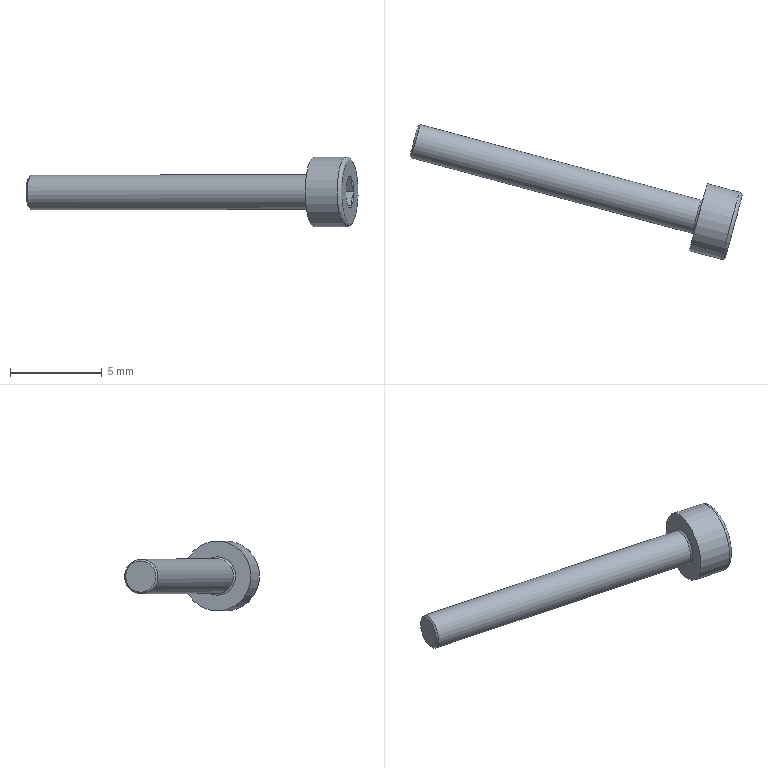Component | NX | GB-T70_1-2000_M2X16 | 1 solid | 27 faces | volume 64 mm3 | plane 15 | cone 8 | cylinder 2 | torus 2 | commonest cylinder face diameters 1.886 x1 3.8 x1